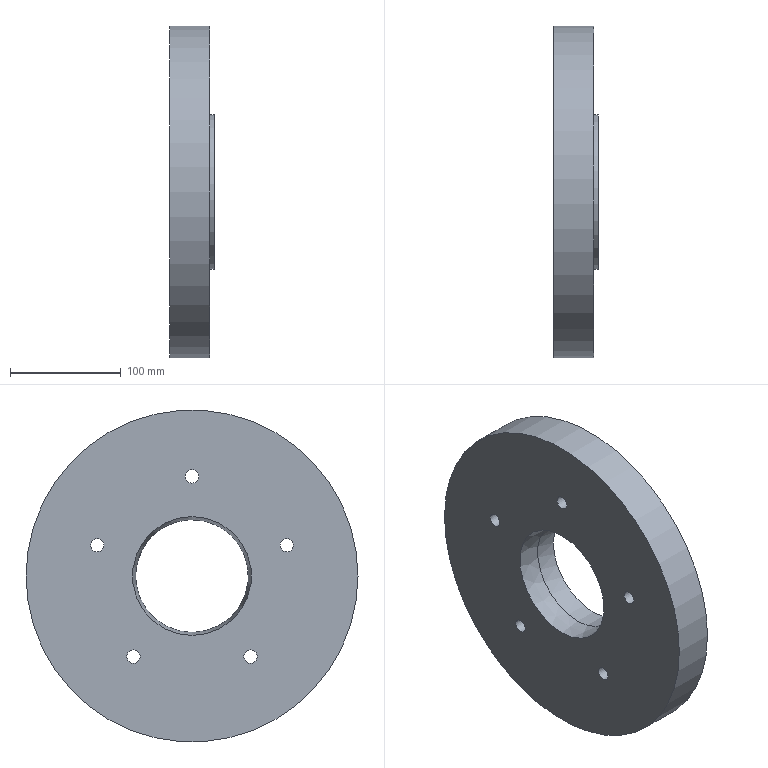Component | NX | ADAPTER_PLATE | 1 solid | 12 faces | box 40 x 300 x 300 mm | volume 2250203 mm3 | cylinder 8 | plane 3 | cone 1 | commonest cylinder face diameters 12 x5 102 x1 300 x1 140 x1
STEP:
#1=CARTESIAN_POINT('',(0.,0.,0.));
#2=DIRECTION('',(0.,0.,1.));
#3=DIRECTION('',(1.,0.,0.));
#4=AXIS2_PLACEMENT_3D('',#1,#2,#3);
#5=CARTESIAN_POINT('',(479.625,0.09065,-51.557));
#6=VERTEX_POINT('',#5);
#7=CARTESIAN_POINT('',(479.625,51.091,-0.557));
#8=VERTEX_POINT('',#7);
#9=CARTESIAN_POINT('',(479.625,0.09065,-0.557));
#10=DIRECTION('',(1.,0.,0.));
#11=DIRECTION('',(0.,1.,-0.));
#12=AXIS2_PLACEMENT_3D('',#9,#10,#11);
#13=CIRCLE('',#12,51.);
#14=CARTESIAN_POINT('',(439.625,0.09065,-0.557));
#15=DIRECTION('',(1.,0.,0.));
#16=DIRECTION('',(0.,0.,-1.));
#17=AXIS2_PLACEMENT_3D('',#14,#15,#16);
#18=CYLINDRICAL_SURFACE('',#17,51.);
#19=CARTESIAN_POINT('',(-4.712,40.));
#20=DIRECTION('',(1.,0.));
#21=VECTOR('',#20,1.);
#22=LINE('',#19,#21);
#23=(GEOMETRIC_REPRESENTATION_CONTEXT(2)PARAMETRIC_REPRESENTATION_CONTEXT()REPRESENTATION_CONTEXT('',''));
#24=DEFINITIONAL_REPRESENTATION('',(#22),#23);
#25=PCURVE('',#18,#24);
#26=CARTESIAN_POINT('',(479.625,0.09065,-0.557));
#27=DIRECTION('',(1.,0.,0.));
#28=DIRECTION('',(0.,0.,-1.));
#29=AXIS2_PLACEMENT_3D('',#26,#27,#28);
#30=PLANE('',#29);
#31=CARTESIAN_POINT('',(0.,0.));
#32=DIRECTION('',(0.,1.));
#33=AXIS2_PLACEMENT_2D('',#31,#32);
#34=CIRCLE('',#33,51.);
#35=(GEOMETRIC_REPRESENTATION_CONTEXT(2)PARAMETRIC_REPRESENTATION_CONTEXT()REPRESENTATION_CONTEXT('',''));
#36=DEFINITIONAL_REPRESENTATION('',(#34),#35);
#37=PCURVE('',#30,#36);
#38=SURFACE_CURVE('',#13,(#25,#37),.PCURVE_S1.);
#39=EDGE_CURVE('',#6,#8,#38,.T.);
#40=ORIENTED_EDGE('',*,*,#39,.F.);
#41=CARTESIAN_POINT('',(459.625,0.09065,-51.557));
#42=VERTEX_POINT('',#41);
#43=CARTESIAN_POINT('',(459.625,0.09065,-51.557));
#44=CARTESIAN_POINT('',(479.625,0.09065,-51.557));
#45=B_SPLINE_CURVE_WITH_KNOTS('',1,(#43,#44),.UNSPECIFIED.,.F.,.F.,(2,2),(20.,40.),.PIECEWISE_BEZIER_KNOTS.);
#46=CARTESIAN_POINT('',(0.,0.));
#47=DIRECTION('',(0.,1.));
#48=VECTOR('',#47,1.);
#49=LINE('',#46,#48);
#50=(GEOMETRIC_REPRESENTATION_CONTEXT(2)PARAMETRIC_REPRESENTATION_CONTEXT()REPRESENTATION_CONTEXT('',''));
#51=DEFINITIONAL_REPRESENTATION('',(#49),#50);
#52=PCURVE('',#18,#51);
#53=CARTESIAN_POINT('',(6.283,0.));
#54=DIRECTION('',(0.,1.));
#55=VECTOR('',#54,1.);
#56=LINE('',#53,#55);
#57=(GEOMETRIC_REPRESENTATION_CONTEXT(2)PARAMETRIC_REPRESENTATION_CONTEXT()REPRESENTATION_CONTEXT('',''));
#58=DEFINITIONAL_REPRESENTATION('',(#56),#57);
#59=PCURVE('',#18,#58);
#60=SEAM_CURVE('',#45,(#52,#59),.PCURVE_S1.);
#61=EDGE_CURVE('',#42,#6,#60,.T.);
#62=ORIENTED_EDGE('',*,*,#61,.F.);
#63=CARTESIAN_POINT('',(459.625,0.09065,-0.557));
#64=DIRECTION('',(1.,0.,0.));
#65=DIRECTION('',(0.,0.,-1.));
#66=AXIS2_PLACEMENT_3D('',#63,#64,#65);
#67=CIRCLE('',#66,51.);
#68=CARTESIAN_POINT('',(0.,20.));
#69=DIRECTION('',(1.,0.));
#70=VECTOR('',#69,1.);
#71=LINE('',#68,#70);
#72=(GEOMETRIC_REPRESENTATION_CONTEXT(2)PARAMETRIC_REPRESENTATION_CONTEXT()REPRESENTATION_CONTEXT('',''));
#73=DEFINITIONAL_REPRESENTATION('',(#71),#72);
#74=PCURVE('',#18,#73);
#75=CARTESIAN_POINT('',(369.452,0.09065,-0.557));
#76=DIRECTION('',(-1.,0.,0.));
#77=DIRECTION('',(0.,0.,1.));
#78=AXIS2_PLACEMENT_3D('',#75,#76,#77);
#79=CONICAL_SURFACE('',#78,63.24,0.1349);
#80=CARTESIAN_POINT('',(9.425,-90.173));
#81=DIRECTION('',(-1.,0.));
#82=VECTOR('',#81,1.);
#83=LINE('',#80,#82);
#84=(GEOMETRIC_REPRESENTATION_CONTEXT(2)PARAMETRIC_REPRESENTATION_CONTEXT()REPRESENTATION_CONTEXT('',''));
#85=DEFINITIONAL_REPRESENTATION('',(#83),#84);
#86=PCURVE('',#79,#85);
#87=SURFACE_CURVE('',#67,(#74,#86),.PCURVE_S1.);
#88=EDGE_CURVE('',#42,#42,#87,.T.);
#89=ORIENTED_EDGE('',*,*,#88,.T.);
#90=ORIENTED_EDGE('',*,*,#61,.T.);
#91=CARTESIAN_POINT('',(479.625,0.09065,-0.557));
#92=DIRECTION('',(1.,0.,0.));
#93=DIRECTION('',(0.,1.,-0.));
#94=AXIS2_PLACEMENT_3D('',#91,#92,#93);
#95=CIRCLE('',#94,51.);
#96=CARTESIAN_POINT('',(1.571,40.));
#97=DIRECTION('',(1.,0.));
#98=VECTOR('',#97,1.);
#99=LINE('',#96,#98);
#100=(GEOMETRIC_REPRESENTATION_CONTEXT(2)PARAMETRIC_REPRESENTATION_CONTEXT()REPRESENTATION_CONTEXT('',''));
#101=DEFINITIONAL_REPRESENTATION('',(#99),#100);
#102=PCURVE('',#18,#101);
#103=CARTESIAN_POINT('',(0.,0.));
#104=DIRECTION('',(0.,1.));
#105=AXIS2_PLACEMENT_2D('',#103,#104);
#106=CIRCLE('',#105,51.);
#107=(GEOMETRIC_REPRESENTATION_CONTEXT(2)PARAMETRIC_REPRESENTATION_CONTEXT()REPRESENTATION_CONTEXT('',''));
#108=DEFINITIONAL_REPRESENTATION('',(#106),#107);
#109=PCURVE('',#30,#108);
#110=SURFACE_CURVE('',#95,(#102,#109),.PCURVE_S1.);
#111=EDGE_CURVE('',#8,#6,#110,.T.);
#112=ORIENTED_EDGE('',*,*,#111,.F.);
#113=EDGE_LOOP('',(#40,#62,#89,#90,#112));
#114=FACE_BOUND('',#113,.F.);
#115=ADVANCED_FACE('',(#114),#18,.F.);
#116=CARTESIAN_POINT('',(475.625,150.091,-0.557));
#117=VERTEX_POINT('',#116);
#118=CARTESIAN_POINT('',(475.625,0.09065,-0.557));
#119=DIRECTION('',(1.,0.,0.));
#120=DIRECTION('',(0.,1.,-0.));
#121=AXIS2_PLACEMENT_3D('',#118,#119,#120);
#122=CIRCLE('',#121,150.);
#123=CARTESIAN_POINT('',(475.625,0.09065,-0.557));
#124=DIRECTION('',(-1.,0.,0.));
#125=DIRECTION('',(0.,0.,1.));
#126=AXIS2_PLACEMENT_3D('',#123,#124,#125);
#127=CYLINDRICAL_SURFACE('',#126,150.);
#128=CARTESIAN_POINT('',(7.854,0.));
#129=DIRECTION('',(-1.,0.));
#130=VECTOR('',#129,1.);
#131=LINE('',#128,#130);
#132=(GEOMETRIC_REPRESENTATION_CONTEXT(2)PARAMETRIC_REPRESENTATION_CONTEXT()REPRESENTATION_CONTEXT('',''));
#133=DEFINITIONAL_REPRESENTATION('',(#131),#132);
#134=PCURVE('',#127,#133);
#135=CARTESIAN_POINT('',(475.625,0.09065,-0.557));
#136=DIRECTION('',(1.,0.,0.));
#137=DIRECTION('',(0.,0.,-1.));
#138=AXIS2_PLACEMENT_3D('',#135,#136,#137);
#139=PLANE('',#138);
#140=CARTESIAN_POINT('',(0.,0.));
#141=DIRECTION('',(0.,1.));
#142=AXIS2_PLACEMENT_2D('',#140,#141);
#143=CIRCLE('',#142,150.);
#144=(GEOMETRIC_REPRESENTATION_CONTEXT(2)PARAMETRIC_REPRESENTATION_CONTEXT()REPRESENTATION_CONTEXT('',''));
#145=DEFINITIONAL_REPRESENTATION('',(#143),#144);
#146=PCURVE('',#139,#145);
#147=SURFACE_CURVE('',#122,(#134,#146),.PCURVE_S1.);
#148=EDGE_CURVE('',#117,#117,#147,.T.);
#149=ORIENTED_EDGE('',*,*,#148,.F.);
#150=CARTESIAN_POINT('',(439.625,150.091,-0.557));
#151=VERTEX_POINT('',#150);
#152=CARTESIAN_POINT('',(475.625,150.091,-0.557));
#153=CARTESIAN_POINT('',(439.625,150.091,-0.557));
#154=B_SPLINE_CURVE_WITH_KNOTS('',1,(#152,#153),.UNSPECIFIED.,.F.,.F.,(2,2),(0.,36.),.PIECEWISE_BEZIER_KNOTS.);
#155=CARTESIAN_POINT('',(7.854,0.));
#156=DIRECTION('',(0.,1.));
#157=VECTOR('',#156,1.);
#158=LINE('',#155,#157);
#159=(GEOMETRIC_REPRESENTATION_CONTEXT(2)PARAMETRIC_REPRESENTATION_CONTEXT()REPRESENTATION_CONTEXT('',''));
#160=DEFINITIONAL_REPRESENTATION('',(#158),#159);
#161=PCURVE('',#127,#160);
#162=CARTESIAN_POINT('',(1.571,0.));
#163=DIRECTION('',(0.,1.));
#164=VECTOR('',#163,1.);
#165=LINE('',#162,#164);
#166=(GEOMETRIC_REPRESENTATION_CONTEXT(2)PARAMETRIC_REPRESENTATION_CONTEXT()REPRESENTATION_CONTEXT('',''));
#167=DEFINITIONAL_REPRESENTATION('',(#165),#166);
#168=PCURVE('',#127,#167);
#169=SEAM_CURVE('',#154,(#161,#168),.PCURVE_S1.);
#170=EDGE_CURVE('',#117,#151,#169,.T.);
#171=ORIENTED_EDGE('',*,*,#170,.T.);
#172=CARTESIAN_POINT('',(439.625,0.09065,-0.557));
#173=DIRECTION('',(1.,0.,0.));
#174=DIRECTION('',(0.,1.,-0.));
#175=AXIS2_PLACEMENT_3D('',#172,#173,#174);
#176=CIRCLE('',#175,150.);
#177=CARTESIAN_POINT('',(7.854,36.));
#178=DIRECTION('',(-1.,0.));
#179=VECTOR('',#178,1.);
#180=LINE('',#177,#179);
#181=(GEOMETRIC_REPRESENTATION_CONTEXT(2)PARAMETRIC_REPRESENTATION_CONTEXT()REPRESENTATION_CONTEXT('',''));
#182=DEFINITIONAL_REPRESENTATION('',(#180),#181);
#183=PCURVE('',#127,#182);
#184=CARTESIAN_POINT('',(439.625,0.09065,-0.557));
#185=DIRECTION('',(1.,0.,0.));
#186=DIRECTION('',(0.,0.,-1.));
#187=AXIS2_PLACEMENT_3D('',#184,#185,#186);
#188=PLANE('',#187);
#189=CARTESIAN_POINT('',(0.,0.));
#190=DIRECTION('',(0.,1.));
#191=AXIS2_PLACEMENT_2D('',#189,#190);
#192=CIRCLE('',#191,150.);
#193=(GEOMETRIC_REPRESENTATION_CONTEXT(2)PARAMETRIC_REPRESENTATION_CONTEXT()REPRESENTATION_CONTEXT('',''));
#194=DEFINITIONAL_REPRESENTATION('',(#192),#193);
#195=PCURVE('',#188,#194);
#196=SURFACE_CURVE('',#176,(#183,#195),.PCURVE_S1.);
#197=EDGE_CURVE('',#151,#151,#196,.T.);
#198=ORIENTED_EDGE('',*,*,#197,.T.);
#199=ORIENTED_EDGE('',*,*,#170,.F.);
#200=EDGE_LOOP('',(#149,#171,#198,#199));
#201=FACE_BOUND('',#200,.T.);
#202=ADVANCED_FACE('',(#201),#127,.T.);
#203=CARTESIAN_POINT('',(475.625,85.686,21.254));
#204=VERTEX_POINT('',#203);
#205=CARTESIAN_POINT('',(475.625,85.686,27.254));
#206=DIRECTION('',(-1.,0.,0.));
#207=DIRECTION('',(0.,0.,-1.));
#208=AXIS2_PLACEMENT_3D('',#205,#206,#207);
#209=CIRCLE('',#208,6.);
#210=CARTESIAN_POINT('',(-21.812,85.595));
#211=CARTESIAN_POINT('',(-21.812,75.203));
#212=CARTESIAN_POINT('',(-30.812,80.399));
#213=CARTESIAN_POINT('',(-39.812,85.595));
#214=CARTESIAN_POINT('',(-30.812,90.791));
#215=CARTESIAN_POINT('',(-21.812,95.987));
#216=CARTESIAN_POINT('',(-21.812,85.595));
#217=(BOUNDED_CURVE()B_SPLINE_CURVE(2,(#210,#211,#212,#213,#214,#215,#216),.UNSPECIFIED.,.T.,.F.)B_SPLINE_CURVE_WITH_KNOTS((1,2,2,2,2,1),(-2.094,0.,2.094,4.189,6.283,8.378),.UNSPECIFIED.)CURVE()GEOMETRIC_REPRESENTATION_ITEM()RATIONAL_B_SPLINE_CURVE((1.,0.5,1.,0.5,1.,0.5,1.))REPRESENTATION_ITEM(''));
#218=(GEOMETRIC_REPRESENTATION_CONTEXT(2)PARAMETRIC_REPRESENTATION_CONTEXT()REPRESENTATION_CONTEXT('',''));
#219=DEFINITIONAL_REPRESENTATION('',(#217),#218);
#220=PCURVE('',#139,#219);
#221=CARTESIAN_POINT('',(475.625,85.686,27.254));
#222=DIRECTION('',(-1.,0.,0.));
#223=DIRECTION('',(0.,0.,1.));
#224=AXIS2_PLACEMENT_3D('',#221,#222,#223);
#225=CYLINDRICAL_SURFACE('',#224,6.);
#226=CARTESIAN_POINT('',(3.142,0.));
#227=DIRECTION('',(1.,0.));
#228=VECTOR('',#227,1.);
#229=LINE('',#226,#228);
#230=(GEOMETRIC_REPRESENTATION_CONTEXT(2)PARAMETRIC_REPRESENTATION_CONTEXT()REPRESENTATION_CONTEXT('',''));
#231=DEFINITIONAL_REPRESENTATION('',(#229),#230);
#232=PCURVE('',#225,#231);
#233=SURFACE_CURVE('',#209,(#220,#232),.PCURVE_S1.);
#234=EDGE_CURVE('',#204,#204,#233,.T.);
#235=ORIENTED_EDGE('',*,*,#234,.T.);
#236=EDGE_LOOP('',(#235));
#237=FACE_BOUND('',#236,.T.);
#238=CARTESIAN_POINT('',(475.625,52.991,-79.369));
#239=VERTEX_POINT('',#238);
#240=CARTESIAN_POINT('',(475.625,52.991,-73.369));
#241=DIRECTION('',(-1.,0.,0.));
#242=DIRECTION('',(0.,0.,-1.));
#243=AXIS2_PLACEMENT_3D('',#240,#241,#242);
#244=CIRCLE('',#243,6.);
#245=CARTESIAN_POINT('',(78.812,52.901));
#246=CARTESIAN_POINT('',(78.812,42.508));
#247=CARTESIAN_POINT('',(69.812,47.705));
#248=CARTESIAN_POINT('',(60.812,52.901));
#249=CARTESIAN_POINT('',(69.812,58.097));
#250=CARTESIAN_POINT('',(78.812,63.293));
#251=CARTESIAN_POINT('',(78.812,52.901));
#252=(BOUNDED_CURVE()B_SPLINE_CURVE(2,(#245,#246,#247,#248,#249,#250,#251),.UNSPECIFIED.,.T.,.F.)B_SPLINE_CURVE_WITH_KNOTS((1,2,2,2,2,1),(-2.094,0.,2.094,4.189,6.283,8.378),.UNSPECIFIED.)CURVE()GEOMETRIC_REPRESENTATION_ITEM()RATIONAL_B_SPLINE_CURVE((1.,0.5,1.,0.5,1.,0.5,1.))REPRESENTATION_ITEM(''));
#253=(GEOMETRIC_REPRESENTATION_CONTEXT(2)PARAMETRIC_REPRESENTATION_CONTEXT()REPRESENTATION_CONTEXT('',''));
#254=DEFINITIONAL_REPRESENTATION('',(#252),#253);
#255=PCURVE('',#139,#254);
#256=CARTESIAN_POINT('',(475.625,52.991,-73.369));
#257=DIRECTION('',(-1.,0.,0.));
#258=DIRECTION('',(0.,0.,1.));
#259=AXIS2_PLACEMENT_3D('',#256,#257,#258);
#260=CYLINDRICAL_SURFACE('',#259,6.);
#261=CARTESIAN_POINT('',(3.142,0.));
#262=DIRECTION('',(1.,0.));
#263=VECTOR('',#262,1.);
#264=LINE('',#261,#263);
#265=(GEOMETRIC_REPRESENTATION_CONTEXT(2)PARAMETRIC_REPRESENTATION_CONTEXT()REPRESENTATION_CONTEXT('',''));
#266=DEFINITIONAL_REPRESENTATION('',(#264),#265);
#267=PCURVE('',#260,#266);
#268=SURFACE_CURVE('',#244,(#255,#267),.PCURVE_S1.);
#269=EDGE_CURVE('',#239,#239,#268,.T.);
#270=ORIENTED_EDGE('',*,*,#269,.T.);
#271=EDGE_LOOP('',(#270));
#272=FACE_BOUND('',#271,.T.);
#273=CARTESIAN_POINT('',(475.625,0.09065,83.443));
#274=VERTEX_POINT('',#273);
#275=CARTESIAN_POINT('',(475.625,0.09065,89.443));
#276=DIRECTION('',(-1.,0.,0.));
#277=DIRECTION('',(0.,0.,-1.));
#278=AXIS2_PLACEMENT_3D('',#275,#276,#277);
#279=CIRCLE('',#278,6.);
#280=CARTESIAN_POINT('',(-84.,0.));
#281=CARTESIAN_POINT('',(-84.,-10.392));
#282=CARTESIAN_POINT('',(-93.,-5.196));
#283=CARTESIAN_POINT('',(-102.,-0.));
#284=CARTESIAN_POINT('',(-93.,5.196));
#285=CARTESIAN_POINT('',(-84.,10.392));
#286=CARTESIAN_POINT('',(-84.,0.));
#287=(BOUNDED_CURVE()B_SPLINE_CURVE(2,(#280,#281,#282,#283,#284,#285,#286),.UNSPECIFIED.,.T.,.F.)B_SPLINE_CURVE_WITH_KNOTS((1,2,2,2,2,1),(-2.094,0.,2.094,4.189,6.283,8.378),.UNSPECIFIED.)CURVE()GEOMETRIC_REPRESENTATION_ITEM()RATIONAL_B_SPLINE_CURVE((1.,0.5,1.,0.5,1.,0.5,1.))REPRESENTATION_ITEM(''));
#288=(GEOMETRIC_REPRESENTATION_CONTEXT(2)PARAMETRIC_REPRESENTATION_CONTEXT()REPRESENTATION_CONTEXT('',''));
#289=DEFINITIONAL_REPRESENTATION('',(#287),#288);
#290=PCURVE('',#139,#289);
#291=CARTESIAN_POINT('',(475.625,0.09065,89.443));
#292=DIRECTION('',(-1.,0.,0.));
#293=DIRECTION('',(0.,0.,1.));
#294=AXIS2_PLACEMENT_3D('',#291,#292,#293);
#295=CYLINDRICAL_SURFACE('',#294,6.);
#296=CARTESIAN_POINT('',(3.142,0.));
#297=DIRECTION('',(1.,0.));
#298=VECTOR('',#297,1.);
#299=LINE('',#296,#298);
#300=(GEOMETRIC_REPRESENTATION_CONTEXT(2)PARAMETRIC_REPRESENTATION_CONTEXT()REPRESENTATION_CONTEXT('',''));
#301=DEFINITIONAL_REPRESENTATION('',(#299),#300);
#302=PCURVE('',#295,#301);
#303=SURFACE_CURVE('',#279,(#290,#302),.PCURVE_S1.);
#304=EDGE_CURVE('',#274,#274,#303,.T.);
#305=ORIENTED_EDGE('',*,*,#304,.T.);
#306=EDGE_LOOP('',(#305));
#307=FACE_BOUND('',#306,.T.);
#308=CARTESIAN_POINT('',(475.625,-52.81,-79.369));
#309=VERTEX_POINT('',#308);
#310=CARTESIAN_POINT('',(475.625,-52.81,-73.369));
#311=DIRECTION('',(-1.,0.,0.));
#312=DIRECTION('',(0.,0.,-1.));
#313=AXIS2_PLACEMENT_3D('',#310,#311,#312);
#314=CIRCLE('',#313,6.);
#315=CARTESIAN_POINT('',(78.812,-52.901));
#316=CARTESIAN_POINT('',(78.812,-63.293));
#317=CARTESIAN_POINT('',(69.812,-58.097));
#318=CARTESIAN_POINT('',(60.812,-52.901));
#319=CARTESIAN_POINT('',(69.812,-47.705));
#320=CARTESIAN_POINT('',(78.812,-42.508));
#321=CARTESIAN_POINT('',(78.812,-52.901));
#322=(BOUNDED_CURVE()B_SPLINE_CURVE(2,(#315,#316,#317,#318,#319,#320,#321),.UNSPECIFIED.,.T.,.F.)B_SPLINE_CURVE_WITH_KNOTS((1,2,2,2,2,1),(-2.094,0.,2.094,4.189,6.283,8.378),.UNSPECIFIED.)CURVE()GEOMETRIC_REPRESENTATION_ITEM()RATIONAL_B_SPLINE_CURVE((1.,0.5,1.,0.5,1.,0.5,1.))REPRESENTATION_ITEM(''));
#323=(GEOMETRIC_REPRESENTATION_CONTEXT(2)PARAMETRIC_REPRESENTATION_CONTEXT()REPRESENTATION_CONTEXT('',''));
#324=DEFINITIONAL_REPRESENTATION('',(#322),#323);
#325=PCURVE('',#139,#324);
#326=CARTESIAN_POINT('',(475.625,-52.81,-73.369));
#327=DIRECTION('',(-1.,0.,0.));
#328=DIRECTION('',(0.,0.,1.));
#329=AXIS2_PLACEMENT_3D('',#326,#327,#328);
#330=CYLINDRICAL_SURFACE('',#329,6.);
#331=CARTESIAN_POINT('',(3.142,0.));
#332=DIRECTION('',(1.,0.));
#333=VECTOR('',#332,1.);
#334=LINE('',#331,#333);
#335=(GEOMETRIC_REPRESENTATION_CONTEXT(2)PARAMETRIC_REPRESENTATION_CONTEXT()REPRESENTATION_CONTEXT('',''));
#336=DEFINITIONAL_REPRESENTATION('',(#334),#335);
#337=PCURVE('',#330,#336);
#338=SURFACE_CURVE('',#314,(#325,#337),.PCURVE_S1.);
#339=EDGE_CURVE('',#309,#309,#338,.T.);
#340=ORIENTED_EDGE('',*,*,#339,.T.);
#341=EDGE_LOOP('',(#340));
#342=FACE_BOUND('',#341,.T.);
#343=CARTESIAN_POINT('',(475.625,-85.504,21.254));
#344=VERTEX_POINT('',#343);
#345=CARTESIAN_POINT('',(475.625,-85.504,27.254));
#346=DIRECTION('',(-1.,0.,0.));
#347=DIRECTION('',(0.,0.,-1.));
#348=AXIS2_PLACEMENT_3D('',#345,#346,#347);
#349=CIRCLE('',#348,6.);
#350=CARTESIAN_POINT('',(-21.812,-85.595));
#351=CARTESIAN_POINT('',(-21.812,-95.987));
#352=CARTESIAN_POINT('',(-30.812,-90.791));
#353=CARTESIAN_POINT('',(-39.812,-85.595));
#354=CARTESIAN_POINT('',(-30.812,-80.399));
#355=CARTESIAN_POINT('',(-21.812,-75.203));
#356=CARTESIAN_POINT('',(-21.812,-85.595));
#357=(BOUNDED_CURVE()B_SPLINE_CURVE(2,(#350,#351,#352,#353,#354,#355,#356),.UNSPECIFIED.,.T.,.F.)B_SPLINE_CURVE_WITH_KNOTS((1,2,2,2,2,1),(-2.094,0.,2.094,4.189,6.283,8.378),.UNSPECIFIED.)CURVE()GEOMETRIC_REPRESENTATION_ITEM()RATIONAL_B_SPLINE_CURVE((1.,0.5,1.,0.5,1.,0.5,1.))REPRESENTATION_ITEM(''));
#358=(GEOMETRIC_REPRESENTATION_CONTEXT(2)PARAMETRIC_REPRESENTATION_CONTEXT()REPRESENTATION_CONTEXT('',''));
#359=DEFINITIONAL_REPRESENTATION('',(#357),#358);
#360=PCURVE('',#139,#359);
#361=CARTESIAN_POINT('',(475.625,-85.504,27.254));
#362=DIRECTION('',(-1.,0.,0.));
#363=DIRECTION('',(0.,0.,1.));
#364=AXIS2_PLACEMENT_3D('',#361,#362,#363);
#365=CYLINDRICAL_SURFACE('',#364,6.);
#366=CARTESIAN_POINT('',(3.142,0.));
#367=DIRECTION('',(1.,0.));
#368=VECTOR('',#367,1.);
#369=LINE('',#366,#368);
#370=(GEOMETRIC_REPRESENTATION_CONTEXT(2)PARAMETRIC_REPRESENTATION_CONTEXT()REPRESENTATION_CONTEXT('',''));
#371=DEFINITIONAL_REPRESENTATION('',(#369),#370);
#372=PCURVE('',#365,#371);
#373=SURFACE_CURVE('',#349,(#360,#372),.PCURVE_S1.);
#374=EDGE_CURVE('',#344,#344,#373,.T.);
#375=ORIENTED_EDGE('',*,*,#374,.T.);
#376=EDGE_LOOP('',(#375));
#377=FACE_BOUND('',#376,.T.);
#378=CARTESIAN_POINT('',(475.625,70.091,-0.557));
#379=VERTEX_POINT('',#378);
#380=CARTESIAN_POINT('',(475.625,0.09065,-0.557));
#381=DIRECTION('',(1.,0.,0.));
#382=DIRECTION('',(0.,1.,-0.));
#383=AXIS2_PLACEMENT_3D('',#380,#381,#382);
#384=CIRCLE('',#383,70.);
#385=CARTESIAN_POINT('',(0.,0.));
#386=DIRECTION('',(0.,1.));
#387=AXIS2_PLACEMENT_2D('',#385,#386);
#388=CIRCLE('',#387,70.);
#389=(GEOMETRIC_REPRESENTATION_CONTEXT(2)PARAMETRIC_REPRESENTATION_CONTEXT()REPRESENTATION_CONTEXT('',''));
#390=DEFINITIONAL_REPRESENTATION('',(#388),#389);
#391=PCURVE('',#139,#390);
#392=CARTESIAN_POINT('',(479.625,0.09065,-0.557));
#393=DIRECTION('',(-1.,0.,0.));
#394=DIRECTION('',(0.,0.,1.));
#395=AXIS2_PLACEMENT_3D('',#392,#393,#394);
#396=CYLINDRICAL_SURFACE('',#395,70.);
#397=CARTESIAN_POINT('',(7.854,4.));
#398=DIRECTION('',(-1.,0.));
#399=VECTOR('',#398,1.);
#400=LINE('',#397,#399);
#401=(GEOMETRIC_REPRESENTATION_CONTEXT(2)PARAMETRIC_REPRESENTATION_CONTEXT()REPRESENTATION_CONTEXT('',''));
#402=DEFINITIONAL_REPRESENTATION('',(#400),#401);
#403=PCURVE('',#396,#402);
#404=SURFACE_CURVE('',#384,(#391,#403),.PCURVE_S1.);
#405=EDGE_CURVE('',#379,#379,#404,.T.);
#406=ORIENTED_EDGE('',*,*,#405,.F.);
#407=EDGE_LOOP('',(#406));
#408=FACE_BOUND('',#407,.T.);
#409=ORIENTED_EDGE('',*,*,#148,.T.);
#410=EDGE_LOOP('',(#409));
#411=FACE_BOUND('',#410,.T.);
#412=ADVANCED_FACE('',(#237,#272,#307,#342,#377,#408,#411),#139,.T.);
#413=CARTESIAN_POINT('',(439.625,0.09065,-54.272));
#414=VERTEX_POINT('',#413);
#415=CARTESIAN_POINT('',(439.625,0.09065,-0.557));
#416=DIRECTION('',(-1.,0.,0.));
#417=DIRECTION('',(0.,0.,-1.));
#418=AXIS2_PLACEMENT_3D('',#415,#416,#417);
#419=CIRCLE('',#418,53.715);
#420=CARTESIAN_POINT('',(53.715,0.));
#421=CARTESIAN_POINT('',(53.715,-93.037));
#422=CARTESIAN_POINT('',(-26.857,-46.518));
#423=CARTESIAN_POINT('',(-107.43,-0.));
#424=CARTESIAN_POINT('',(-26.857,46.518));
#425=CARTESIAN_POINT('',(53.715,93.037));
#426=CARTESIAN_POINT('',(53.715,0.));
#427=(BOUNDED_CURVE()B_SPLINE_CURVE(2,(#420,#421,#422,#423,#424,#425,#426),.UNSPECIFIED.,.T.,.F.)B_SPLINE_CURVE_WITH_KNOTS((1,2,2,2,2,1),(-2.094,0.,2.094,4.189,6.283,8.378),.UNSPECIFIED.)CURVE()GEOMETRIC_REPRESENTATION_ITEM()RATIONAL_B_SPLINE_CURVE((1.,0.5,1.,0.5,1.,0.5,1.))REPRESENTATION_ITEM(''));
#428=(GEOMETRIC_REPRESENTATION_CONTEXT(2)PARAMETRIC_REPRESENTATION_CONTEXT()REPRESENTATION_CONTEXT('',''));
#429=DEFINITIONAL_REPRESENTATION('',(#427),#428);
#430=PCURVE('',#188,#429);
#431=CARTESIAN_POINT('',(3.142,-70.173));
#432=DIRECTION('',(1.,0.));
#433=VECTOR('',#432,1.);
#434=LINE('',#431,#433);
#435=(GEOMETRIC_REPRESENTATION_CONTEXT(2)PARAMETRIC_REPRESENTATION_CONTEXT()REPRESENTATION_CONTEXT('',''));
#436=DEFINITIONAL_REPRESENTATION('',(#434),#435);
#437=PCURVE('',#79,#436);
#438=SURFACE_CURVE('',#419,(#430,#437),.PCURVE_S1.);
#439=EDGE_CURVE('',#414,#414,#438,.T.);
#440=ORIENTED_EDGE('',*,*,#439,.F.);
#441=EDGE_LOOP('',(#440));
#442=FACE_BOUND('',#441,.T.);
#443=CARTESIAN_POINT('',(439.625,85.686,21.254));
#444=VERTEX_POINT('',#443);
#445=CARTESIAN_POINT('',(439.625,85.686,27.254));
#446=DIRECTION('',(1.,0.,0.));
#447=DIRECTION('',(0.,0.,-1.));
#448=AXIS2_PLACEMENT_3D('',#445,#446,#447);
#449=CIRCLE('',#448,6.);
#450=CARTESIAN_POINT('',(-27.812,85.595));
#451=DIRECTION('',(1.,0.));
#452=AXIS2_PLACEMENT_2D('',#450,#451);
#453=CIRCLE('',#452,6.);
#454=(GEOMETRIC_REPRESENTATION_CONTEXT(2)PARAMETRIC_REPRESENTATION_CONTEXT()REPRESENTATION_CONTEXT('',''));
#455=DEFINITIONAL_REPRESENTATION('',(#453),#454);
#456=PCURVE('',#188,#455);
#457=CARTESIAN_POINT('',(9.425,36.));
#458=DIRECTION('',(-1.,0.));
#459=VECTOR('',#458,1.);
#460=LINE('',#457,#459);
#461=(GEOMETRIC_REPRESENTATION_CONTEXT(2)PARAMETRIC_REPRESENTATION_CONTEXT()REPRESENTATION_CONTEXT('',''));
#462=DEFINITIONAL_REPRESENTATION('',(#460),#461);
#463=PCURVE('',#225,#462);
#464=SURFACE_CURVE('',#449,(#456,#463),.PCURVE_S1.);
#465=EDGE_CURVE('',#444,#444,#464,.T.);
#466=ORIENTED_EDGE('',*,*,#465,.T.);
#467=EDGE_LOOP('',(#466));
#468=FACE_BOUND('',#467,.T.);
#469=CARTESIAN_POINT('',(439.625,52.991,-79.369));
#470=VERTEX_POINT('',#469);
#471=CARTESIAN_POINT('',(439.625,52.991,-73.369));
#472=DIRECTION('',(1.,0.,0.));
#473=DIRECTION('',(0.,0.,-1.));
#474=AXIS2_PLACEMENT_3D('',#471,#472,#473);
#475=CIRCLE('',#474,6.);
#476=CARTESIAN_POINT('',(72.812,52.901));
#477=DIRECTION('',(1.,0.));
#478=AXIS2_PLACEMENT_2D('',#476,#477);
#479=CIRCLE('',#478,6.);
#480=(GEOMETRIC_REPRESENTATION_CONTEXT(2)PARAMETRIC_REPRESENTATION_CONTEXT()REPRESENTATION_CONTEXT('',''));
#481=DEFINITIONAL_REPRESENTATION('',(#479),#480);
#482=PCURVE('',#188,#481);
#483=CARTESIAN_POINT('',(9.425,36.));
#484=DIRECTION('',(-1.,0.));
#485=VECTOR('',#484,1.);
#486=LINE('',#483,#485);
#487=(GEOMETRIC_REPRESENTATION_CONTEXT(2)PARAMETRIC_REPRESENTATION_CONTEXT()REPRESENTATION_CONTEXT('',''));
#488=DEFINITIONAL_REPRESENTATION('',(#486),#487);
#489=PCURVE('',#260,#488);
#490=SURFACE_CURVE('',#475,(#482,#489),.PCURVE_S1.);
#491=EDGE_CURVE('',#470,#470,#490,.T.);
#492=ORIENTED_EDGE('',*,*,#491,.T.);
#493=EDGE_LOOP('',(#492));
#494=FACE_BOUND('',#493,.T.);
#495=CARTESIAN_POINT('',(439.625,0.09065,83.443));
#496=VERTEX_POINT('',#495);
#497=CARTESIAN_POINT('',(439.625,0.09065,89.443));
#498=DIRECTION('',(1.,0.,0.));
#499=DIRECTION('',(0.,0.,-1.));
#500=AXIS2_PLACEMENT_3D('',#497,#498,#499);
#501=CIRCLE('',#500,6.);
#502=CARTESIAN_POINT('',(-90.,0.));
#503=DIRECTION('',(1.,0.));
#504=AXIS2_PLACEMENT_2D('',#502,#503);
#505=CIRCLE('',#504,6.);
#506=(GEOMETRIC_REPRESENTATION_CONTEXT(2)PARAMETRIC_REPRESENTATION_CONTEXT()REPRESENTATION_CONTEXT('',''));
#507=DEFINITIONAL_REPRESENTATION('',(#505),#506);
#508=PCURVE('',#188,#507);
#509=CARTESIAN_POINT('',(9.425,36.));
#510=DIRECTION('',(-1.,0.));
#511=VECTOR('',#510,1.);
#512=LINE('',#509,#511);
#513=(GEOMETRIC_REPRESENTATION_CONTEXT(2)PARAMETRIC_REPRESENTATION_CONTEXT()REPRESENTATION_CONTEXT('',''));
#514=DEFINITIONAL_REPRESENTATION('',(#512),#513);
#515=PCURVE('',#295,#514);
#516=SURFACE_CURVE('',#501,(#508,#515),.PCURVE_S1.);
#517=EDGE_CURVE('',#496,#496,#516,.T.);
#518=ORIENTED_EDGE('',*,*,#517,.T.);
#519=EDGE_LOOP('',(#518));
#520=FACE_BOUND('',#519,.T.);
#521=CARTESIAN_POINT('',(439.625,-52.81,-79.369));
#522=VERTEX_POINT('',#521);
#523=CARTESIAN_POINT('',(439.625,-52.81,-73.369));
#524=DIRECTION('',(1.,0.,0.));
#525=DIRECTION('',(0.,0.,-1.));
#526=AXIS2_PLACEMENT_3D('',#523,#524,#525);
#527=CIRCLE('',#526,6.);
#528=CARTESIAN_POINT('',(72.812,-52.901));
#529=DIRECTION('',(1.,0.));
#530=AXIS2_PLACEMENT_2D('',#528,#529);
#531=CIRCLE('',#530,6.);
#532=(GEOMETRIC_REPRESENTATION_CONTEXT(2)PARAMETRIC_REPRESENTATION_CONTEXT()REPRESENTATION_CONTEXT('',''));
#533=DEFINITIONAL_REPRESENTATION('',(#531),#532);
#534=PCURVE('',#188,#533);
#535=CARTESIAN_POINT('',(9.425,36.));
#536=DIRECTION('',(-1.,0.));
#537=VECTOR('',#536,1.);
#538=LINE('',#535,#537);
#539=(GEOMETRIC_REPRESENTATION_CONTEXT(2)PARAMETRIC_REPRESENTATION_CONTEXT()REPRESENTATION_CONTEXT('',''));
#540=DEFINITIONAL_REPRESENTATION('',(#538),#539);
#541=PCURVE('',#330,#540);
#542=SURFACE_CURVE('',#527,(#534,#541),.PCURVE_S1.);
#543=EDGE_CURVE('',#522,#522,#542,.T.);
#544=ORIENTED_EDGE('',*,*,#543,.T.);
#545=EDGE_LOOP('',(#544));
#546=FACE_BOUND('',#545,.T.);
#547=CARTESIAN_POINT('',(439.625,-85.504,21.254));
#548=VERTEX_POINT('',#547);
#549=CARTESIAN_POINT('',(439.625,-85.504,27.254));
#550=DIRECTION('',(1.,0.,0.));
#551=DIRECTION('',(0.,0.,-1.));
#552=AXIS2_PLACEMENT_3D('',#549,#550,#551);
#553=CIRCLE('',#552,6.);
#554=CARTESIAN_POINT('',(-27.812,-85.595));
#555=DIRECTION('',(1.,0.));
#556=AXIS2_PLACEMENT_2D('',#554,#555);
#557=CIRCLE('',#556,6.);
#558=(GEOMETRIC_REPRESENTATION_CONTEXT(2)PARAMETRIC_REPRESENTATION_CONTEXT()REPRESENTATION_CONTEXT('',''));
#559=DEFINITIONAL_REPRESENTATION('',(#557),#558);
#560=PCURVE('',#188,#559);
#561=CARTESIAN_POINT('',(9.425,36.));
#562=DIRECTION('',(-1.,0.));
#563=VECTOR('',#562,1.);
#564=LINE('',#561,#563);
#565=(GEOMETRIC_REPRESENTATION_CONTEXT(2)PARAMETRIC_REPRESENTATION_CONTEXT()REPRESENTATION_CONTEXT('',''));
#566=DEFINITIONAL_REPRESENTATION('',(#564),#565);
#567=PCURVE('',#365,#566);
#568=SURFACE_CURVE('',#553,(#560,#567),.PCURVE_S1.);
#569=EDGE_CURVE('',#548,#548,#568,.T.);
#570=ORIENTED_EDGE('',*,*,#569,.T.);
#571=EDGE_LOOP('',(#570));
#572=FACE_BOUND('',#571,.T.);
#573=ORIENTED_EDGE('',*,*,#197,.F.);
#574=EDGE_LOOP('',(#573));
#575=FACE_BOUND('',#574,.T.);
#576=ADVANCED_FACE('',(#442,#468,#494,#520,#546,#572,#575),#188,.F.);
#577=CARTESIAN_POINT('',(479.625,70.091,-0.557));
#578=VERTEX_POINT('',#577);
#579=CARTESIAN_POINT('',(479.625,0.09065,-0.557));
#580=DIRECTION('',(1.,0.,0.));
#581=DIRECTION('',(0.,1.,-0.));
#582=AXIS2_PLACEMENT_3D('',#579,#580,#581);
#583=CIRCLE('',#582,70.);
#584=CARTESIAN_POINT('',(7.854,0.));
#585=DIRECTION('',(-1.,0.));
#586=VECTOR('',#585,1.);
#587=LINE('',#584,#586);
#588=(GEOMETRIC_REPRESENTATION_CONTEXT(2)PARAMETRIC_REPRESENTATION_CONTEXT()REPRESENTATION_CONTEXT('',''));
#589=DEFINITIONAL_REPRESENTATION('',(#587),#588);
#590=PCURVE('',#396,#589);
#591=CARTESIAN_POINT('',(0.,0.));
#592=DIRECTION('',(0.,1.));
#593=AXIS2_PLACEMENT_2D('',#591,#592);
#594=CIRCLE('',#593,70.);
#595=(GEOMETRIC_REPRESENTATION_CONTEXT(2)PARAMETRIC_REPRESENTATION_CONTEXT()REPRESENTATION_CONTEXT('',''));
#596=DEFINITIONAL_REPRESENTATION('',(#594),#595);
#597=PCURVE('',#30,#596);
#598=SURFACE_CURVE('',#583,(#590,#597),.PCURVE_S1.);
#599=EDGE_CURVE('',#578,#578,#598,.T.);
#600=ORIENTED_EDGE('',*,*,#599,.F.);
#601=CARTESIAN_POINT('',(479.625,70.091,-0.557));
#602=CARTESIAN_POINT('',(475.625,70.091,-0.557));
#603=B_SPLINE_CURVE_WITH_KNOTS('',1,(#601,#602),.UNSPECIFIED.,.F.,.F.,(2,2),(0.,4.),.PIECEWISE_BEZIER_KNOTS.);
#604=CARTESIAN_POINT('',(7.854,0.));
#605=DIRECTION('',(0.,1.));
#606=VECTOR('',#605,1.);
#607=LINE('',#604,#606);
#608=(GEOMETRIC_REPRESENTATION_CONTEXT(2)PARAMETRIC_REPRESENTATION_CONTEXT()REPRESENTATION_CONTEXT('',''));
#609=DEFINITIONAL_REPRESENTATION('',(#607),#608);
#610=PCURVE('',#396,#609);
#611=CARTESIAN_POINT('',(1.571,0.));
#612=DIRECTION('',(0.,1.));
#613=VECTOR('',#612,1.);
#614=LINE('',#611,#613);
#615=(GEOMETRIC_REPRESENTATION_CONTEXT(2)PARAMETRIC_REPRESENTATION_CONTEXT()REPRESENTATION_CONTEXT('',''));
#616=DEFINITIONAL_REPRESENTATION('',(#614),#615);
#617=PCURVE('',#396,#616);
#618=SEAM_CURVE('',#603,(#610,#617),.PCURVE_S1.);
#619=EDGE_CURVE('',#578,#379,#618,.T.);
#620=ORIENTED_EDGE('',*,*,#619,.T.);
#621=ORIENTED_EDGE('',*,*,#405,.T.);
#622=ORIENTED_EDGE('',*,*,#619,.F.);
#623=EDGE_LOOP('',(#600,#620,#621,#622));
#624=FACE_BOUND('',#623,.T.);
#625=ADVANCED_FACE('',(#624),#396,.T.);
#626=ORIENTED_EDGE('',*,*,#111,.F.);
#627=ORIENTED_EDGE('',*,*,#39,.F.);
#628=EDGE_LOOP('',(#626,#627));
#629=FACE_BOUND('',#628,.T.);
#630=ORIENTED_EDGE('',*,*,#599,.T.);
#631=EDGE_LOOP('',(#630));
#632=FACE_BOUND('',#631,.T.);
#633=ADVANCED_FACE('',(#629,#632),#30,.T.);
#634=ORIENTED_EDGE('',*,*,#374,.T.);
#635=CARTESIAN_POINT('',(475.625,-85.504,21.254));
#636=CARTESIAN_POINT('',(439.625,-85.504,21.254));
#637=B_SPLINE_CURVE_WITH_KNOTS('',1,(#635,#636),.UNSPECIFIED.,.F.,.F.,(2,2),(0.,36.),.PIECEWISE_BEZIER_KNOTS.);
#638=CARTESIAN_POINT('',(9.425,0.));
#639=DIRECTION('',(0.,1.));
#640=VECTOR('',#639,1.);
#641=LINE('',#638,#640);
#642=(GEOMETRIC_REPRESENTATION_CONTEXT(2)PARAMETRIC_REPRESENTATION_CONTEXT()REPRESENTATION_CONTEXT('',''));
#643=DEFINITIONAL_REPRESENTATION('',(#641),#642);
#644=PCURVE('',#365,#643);
#645=CARTESIAN_POINT('',(3.142,0.));
#646=DIRECTION('',(0.,1.));
#647=VECTOR('',#646,1.);
#648=LINE('',#645,#647);
#649=(GEOMETRIC_REPRESENTATION_CONTEXT(2)PARAMETRIC_REPRESENTATION_CONTEXT()REPRESENTATION_CONTEXT('',''));
#650=DEFINITIONAL_REPRESENTATION('',(#648),#649);
#651=PCURVE('',#365,#650);
#652=SEAM_CURVE('',#637,(#644,#651),.PCURVE_S1.);
#653=EDGE_CURVE('',#344,#548,#652,.T.);
#654=ORIENTED_EDGE('',*,*,#653,.T.);
#655=ORIENTED_EDGE('',*,*,#569,.T.);
#656=ORIENTED_EDGE('',*,*,#653,.F.);
#657=EDGE_LOOP('',(#634,#654,#655,#656));
#658=FACE_BOUND('',#657,.F.);
#659=ADVANCED_FACE('',(#658),#365,.F.);
#660=ORIENTED_EDGE('',*,*,#339,.T.);
#661=CARTESIAN_POINT('',(475.625,-52.81,-79.369));
#662=CARTESIAN_POINT('',(439.625,-52.81,-79.369));
#663=B_SPLINE_CURVE_WITH_KNOTS('',1,(#661,#662),.UNSPECIFIED.,.F.,.F.,(2,2),(0.,36.),.PIECEWISE_BEZIER_KNOTS.);
#664=CARTESIAN_POINT('',(9.425,0.));
#665=DIRECTION('',(0.,1.));
#666=VECTOR('',#665,1.);
#667=LINE('',#664,#666);
#668=(GEOMETRIC_REPRESENTATION_CONTEXT(2)PARAMETRIC_REPRESENTATION_CONTEXT()REPRESENTATION_CONTEXT('',''));
#669=DEFINITIONAL_REPRESENTATION('',(#667),#668);
#670=PCURVE('',#330,#669);
#671=CARTESIAN_POINT('',(3.142,0.));
#672=DIRECTION('',(0.,1.));
#673=VECTOR('',#672,1.);
#674=LINE('',#671,#673);
#675=(GEOMETRIC_REPRESENTATION_CONTEXT(2)PARAMETRIC_REPRESENTATION_CONTEXT()REPRESENTATION_CONTEXT('',''));
#676=DEFINITIONAL_REPRESENTATION('',(#674),#675);
#677=PCURVE('',#330,#676);
#678=SEAM_CURVE('',#663,(#670,#677),.PCURVE_S1.);
#679=EDGE_CURVE('',#309,#522,#678,.T.);
#680=ORIENTED_EDGE('',*,*,#679,.T.);
#681=ORIENTED_EDGE('',*,*,#543,.T.);
#682=ORIENTED_EDGE('',*,*,#679,.F.);
#683=EDGE_LOOP('',(#660,#680,#681,#682));
#684=FACE_BOUND('',#683,.F.);
#685=ADVANCED_FACE('',(#684),#330,.F.);
#686=ORIENTED_EDGE('',*,*,#304,.T.);
#687=CARTESIAN_POINT('',(475.625,0.09065,83.443));
#688=CARTESIAN_POINT('',(439.625,0.09065,83.443));
#689=B_SPLINE_CURVE_WITH_KNOTS('',1,(#687,#688),.UNSPECIFIED.,.F.,.F.,(2,2),(0.,36.),.PIECEWISE_BEZIER_KNOTS.);
#690=CARTESIAN_POINT('',(9.425,0.));
#691=DIRECTION('',(0.,1.));
#692=VECTOR('',#691,1.);
#693=LINE('',#690,#692);
#694=(GEOMETRIC_REPRESENTATION_CONTEXT(2)PARAMETRIC_REPRESENTATION_CONTEXT()REPRESENTATION_CONTEXT('',''));
#695=DEFINITIONAL_REPRESENTATION('',(#693),#694);
#696=PCURVE('',#295,#695);
#697=CARTESIAN_POINT('',(3.142,0.));
#698=DIRECTION('',(0.,1.));
#699=VECTOR('',#698,1.);
#700=LINE('',#697,#699);
#701=(GEOMETRIC_REPRESENTATION_CONTEXT(2)PARAMETRIC_REPRESENTATION_CONTEXT()REPRESENTATION_CONTEXT('',''));
#702=DEFINITIONAL_REPRESENTATION('',(#700),#701);
#703=PCURVE('',#295,#702);
#704=SEAM_CURVE('',#689,(#696,#703),.PCURVE_S1.);
#705=EDGE_CURVE('',#274,#496,#704,.T.);
#706=ORIENTED_EDGE('',*,*,#705,.T.);
#707=ORIENTED_EDGE('',*,*,#517,.T.);
#708=ORIENTED_EDGE('',*,*,#705,.F.);
#709=EDGE_LOOP('',(#686,#706,#707,#708));
#710=FACE_BOUND('',#709,.F.);
#711=ADVANCED_FACE('',(#710),#295,.F.);
#712=ORIENTED_EDGE('',*,*,#269,.T.);
#713=CARTESIAN_POINT('',(475.625,52.991,-79.369));
#714=CARTESIAN_POINT('',(439.625,52.991,-79.369));
#715=B_SPLINE_CURVE_WITH_KNOTS('',1,(#713,#714),.UNSPECIFIED.,.F.,.F.,(2,2),(0.,36.),.PIECEWISE_BEZIER_KNOTS.);
#716=CARTESIAN_POINT('',(9.425,0.));
#717=DIRECTION('',(0.,1.));
#718=VECTOR('',#717,1.);
#719=LINE('',#716,#718);
#720=(GEOMETRIC_REPRESENTATION_CONTEXT(2)PARAMETRIC_REPRESENTATION_CONTEXT()REPRESENTATION_CONTEXT('',''));
#721=DEFINITIONAL_REPRESENTATION('',(#719),#720);
#722=PCURVE('',#260,#721);
#723=CARTESIAN_POINT('',(3.142,0.));
#724=DIRECTION('',(0.,1.));
#725=VECTOR('',#724,1.);
#726=LINE('',#723,#725);
#727=(GEOMETRIC_REPRESENTATION_CONTEXT(2)PARAMETRIC_REPRESENTATION_CONTEXT()REPRESENTATION_CONTEXT('',''));
#728=DEFINITIONAL_REPRESENTATION('',(#726),#727);
#729=PCURVE('',#260,#728);
#730=SEAM_CURVE('',#715,(#722,#729),.PCURVE_S1.);
#731=EDGE_CURVE('',#239,#470,#730,.T.);
#732=ORIENTED_EDGE('',*,*,#731,.T.);
#733=ORIENTED_EDGE('',*,*,#491,.T.);
#734=ORIENTED_EDGE('',*,*,#731,.F.);
#735=EDGE_LOOP('',(#712,#732,#733,#734));
#736=FACE_BOUND('',#735,.F.);
#737=ADVANCED_FACE('',(#736),#260,.F.);
#738=ORIENTED_EDGE('',*,*,#234,.T.);
#739=CARTESIAN_POINT('',(475.625,85.686,21.254));
#740=CARTESIAN_POINT('',(439.625,85.686,21.254));
#741=B_SPLINE_CURVE_WITH_KNOTS('',1,(#739,#740),.UNSPECIFIED.,.F.,.F.,(2,2),(0.,36.),.PIECEWISE_BEZIER_KNOTS.);
#742=CARTESIAN_POINT('',(9.425,0.));
#743=DIRECTION('',(0.,1.));
#744=VECTOR('',#743,1.);
#745=LINE('',#742,#744);
#746=(GEOMETRIC_REPRESENTATION_CONTEXT(2)PARAMETRIC_REPRESENTATION_CONTEXT()REPRESENTATION_CONTEXT('',''));
#747=DEFINITIONAL_REPRESENTATION('',(#745),#746);
#748=PCURVE('',#225,#747);
#749=CARTESIAN_POINT('',(3.142,0.));
#750=DIRECTION('',(0.,1.));
#751=VECTOR('',#750,1.);
#752=LINE('',#749,#751);
#753=(GEOMETRIC_REPRESENTATION_CONTEXT(2)PARAMETRIC_REPRESENTATION_CONTEXT()REPRESENTATION_CONTEXT('',''));
#754=DEFINITIONAL_REPRESENTATION('',(#752),#753);
#755=PCURVE('',#225,#754);
#756=SEAM_CURVE('',#741,(#748,#755),.PCURVE_S1.);
#757=EDGE_CURVE('',#204,#444,#756,.T.);
#758=ORIENTED_EDGE('',*,*,#757,.T.);
#759=ORIENTED_EDGE('',*,*,#465,.T.);
#760=ORIENTED_EDGE('',*,*,#757,.F.);
#761=EDGE_LOOP('',(#738,#758,#759,#760));
#762=FACE_BOUND('',#761,.F.);
#763=ADVANCED_FACE('',(#762),#225,.F.);
#764=ORIENTED_EDGE('',*,*,#88,.F.);
#765=CARTESIAN_POINT('',(459.625,0.09065,-51.557));
#766=CARTESIAN_POINT('',(439.625,0.09065,-54.272));
#767=B_SPLINE_CURVE_WITH_KNOTS('',1,(#765,#766),.UNSPECIFIED.,.F.,.F.,(2,2),(-91.,-70.817),.PIECEWISE_BEZIER_KNOTS.);
#768=CARTESIAN_POINT('',(9.425,0.));
#769=DIRECTION('',(0.,1.));
#770=VECTOR('',#769,1.);
#771=LINE('',#768,#770);
#772=(GEOMETRIC_REPRESENTATION_CONTEXT(2)PARAMETRIC_REPRESENTATION_CONTEXT()REPRESENTATION_CONTEXT('',''));
#773=DEFINITIONAL_REPRESENTATION('',(#771),#772);
#774=PCURVE('',#79,#773);
#775=CARTESIAN_POINT('',(3.142,0.));
#776=DIRECTION('',(0.,1.));
#777=VECTOR('',#776,1.);
#778=LINE('',#775,#777);
#779=(GEOMETRIC_REPRESENTATION_CONTEXT(2)PARAMETRIC_REPRESENTATION_CONTEXT()REPRESENTATION_CONTEXT('',''));
#780=DEFINITIONAL_REPRESENTATION('',(#778),#779);
#781=PCURVE('',#79,#780);
#782=SEAM_CURVE('',#767,(#774,#781),.PCURVE_S1.);
#783=EDGE_CURVE('',#42,#414,#782,.T.);
#784=ORIENTED_EDGE('',*,*,#783,.T.);
#785=ORIENTED_EDGE('',*,*,#439,.F.);
#786=ORIENTED_EDGE('',*,*,#783,.F.);
#787=EDGE_LOOP('',(#764,#784,#785,#786));
#788=FACE_BOUND('',#787,.F.);
#789=ADVANCED_FACE('',(#788),#79,.F.);
#790=CLOSED_SHELL('',(#115,#202,#412,#576,#625,#633,#659,#685,#711,#737,#763,#789));
#791=MANIFOLD_SOLID_BREP('',#790);
#792=(LENGTH_UNIT()NAMED_UNIT(*)SI_UNIT(.MILLI.,.METRE.));
#793=UNCERTAINTY_MEASURE_WITH_UNIT(LENGTH_MEASURE(0.00001),#792,'','');
#794=(NAMED_UNIT(*)PLANE_ANGLE_UNIT()SI_UNIT($,.RADIAN.));
#795=(NAMED_UNIT(*)SI_UNIT($,.STERADIAN.)SOLID_ANGLE_UNIT());
#796=(GEOMETRIC_REPRESENTATION_CONTEXT(3)GLOBAL_UNCERTAINTY_ASSIGNED_CONTEXT((#793))GLOBAL_UNIT_ASSIGNED_CONTEXT((#792,#794,#795))REPRESENTATION_CONTEXT('',''));
#797=ADVANCED_BREP_SHAPE_REPRESENTATION('',(#4,#791),#796);